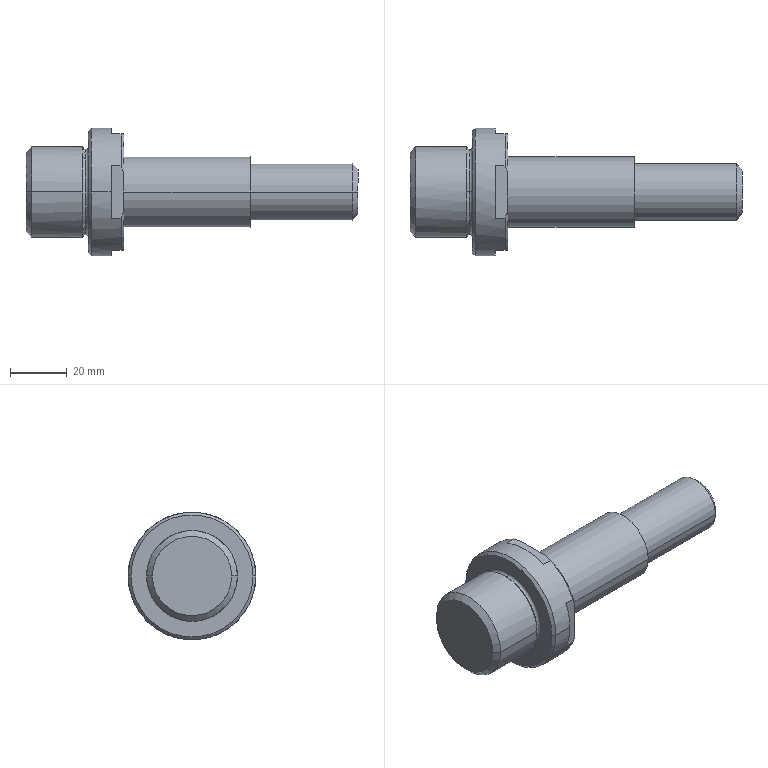Component | SolidWorks | FE5-225--a_b-1 | 1 solid | 35 faces | box 117 x 45 x 45 mm | volume 70338 mm3 | plane 13 | cone 10 | cylinder 8 | torus 4 | commonest cylinder face diameters 32 x2 20 x2 25 x2 45 x2
build123d program:
from build123d import *

# Parameters (mm, degrees)
SKETCH2_R       = 1
CHAMFER2_1_SIZE = 2
CHAMFER1_1_SIZE = 1
SKETCH3_W       = 30
SKETCH3_H       = 5
SKETCH3_W_2     = 5
SKETCH3_H_2     = 30
EXTRUDE1_DEPTH  = 4.5


with BuildPart() as part:
    # Sketch1 → Revolve1 (revolve)
    with BuildSketch(Plane(origin=(0, 0, 0), x_dir=(0, 0, -1), z_dir=(1, 0, 0))):
        Polygon((-117, 0), (-117, 16), (-95, 16), (-95, 22.5), (-82.5, 22.5), (-82.5, 12.5), (-38, 12.5), (-38, 10), (0, 10), (0, 0), align=None)
    revolve(axis=Axis((0, 0, 0), (0, 0, 1)))

    # Sketch2 → Cut-Revolve1 (revolve, cut)
    with BuildSketch(Plane(origin=(0, 0, 0), x_dir=(0, 0, -1), z_dir=(1, 0, 0)), mode=Mode.PRIVATE) as cut_revolve1_sk:
        with Locations((-96, 16)):
            Circle(SKETCH2_R)
    revolve(cut_revolve1_sk.sketch.rotate(Axis((0, 0, 0), (0, 0, 1)), 90), axis=Axis((0, 0, 0), (0, 0, 1)), mode=Mode.SUBTRACT)

    # Chamfer2-1
    chamfer2_1_edges = [part.edges().sort_by_distance(p)[0] for p in [
        (0, -16, 117),
        (0, -10, 0),
    ]]
    chamfer(chamfer2_1_edges, length=CHAMFER2_1_SIZE)

    # Chamfer1-1
    chamfer1_1_edges = [part.edges().sort_by_distance(p)[0] for p in [
        (0, -22.5, 82.5),
        (0, -22.5, 95),
    ]]
    chamfer(chamfer1_1_edges, length=CHAMFER1_1_SIZE)

    # Sketch3 → Extrude1 (cut)
    with BuildSketch(Plane(origin=(0, 0, 82.5), x_dir=(-1, 0, 0), z_dir=(0, 0, -1))):
        with Locations((0, 23)):
            Rectangle(SKETCH3_W, SKETCH3_H)
        with Locations((23, 0)):
            Rectangle(SKETCH3_W_2, SKETCH3_H_2)
        with Locations((-23, 0)):
            Rectangle(SKETCH3_W_2, SKETCH3_H_2)
        with Locations((0, -23)):
            Rectangle(SKETCH3_W, SKETCH3_H)
    extrude(amount=-EXTRUDE1_DEPTH, mode=Mode.SUBTRACT)


solid = part.part

# Placed as in the assembly
solid = solid.moved(Location((102, 81, -524), (0, -90, 0)))
STEP:
#1=COLOUR_RGB('',0.7922,0.8196,0.9333);
#2=FILL_AREA_STYLE_COLOUR('',#1);
#3=FILL_AREA_STYLE('',(#2));
#4=SURFACE_STYLE_FILL_AREA(#3);
#5=SURFACE_SIDE_STYLE('',(#4));
#6=SURFACE_STYLE_USAGE(.BOTH.,#5);
#7=PRESENTATION_STYLE_ASSIGNMENT((#6));
#8=CARTESIAN_POINT('',(0.2756,3.189,-21.26));
#9=VERTEX_POINT('',#8);
#10=CARTESIAN_POINT('',(0.2362,3.189,-21.22));
#11=VERTEX_POINT('',#10);
#12=CARTESIAN_POINT('',(0.2362,3.189,-21.26));
#13=DIRECTION('',(-0.,-1.,-0.));
#14=DIRECTION('',(1.,0.,0.));
#15=AXIS2_PLACEMENT_3D('',#12,#13,#14);
#16=CIRCLE('',#15,0.03937);
#17=EDGE_CURVE('',#9,#11,#16,.T.);
#18=ORIENTED_EDGE('',*,*,#17,.T.);
#19=CARTESIAN_POINT('',(0.2362,3.189,-20.039));
#20=VERTEX_POINT('',#19);
#21=CARTESIAN_POINT('',(0.2362,3.189,-20.63));
#22=DIRECTION('',(1.,-0.,-0.));
#23=DIRECTION('',(-0.,0.,-1.));
#24=AXIS2_PLACEMENT_3D('',#21,#22,#23);
#25=CIRCLE('',#24,0.5906);
#26=EDGE_CURVE('',#11,#20,#25,.T.);
#27=ORIENTED_EDGE('',*,*,#26,.T.);
#28=CARTESIAN_POINT('',(0.2756,3.189,-20.));
#29=VERTEX_POINT('',#28);
#30=CARTESIAN_POINT('',(0.2362,3.189,-20.));
#31=DIRECTION('',(0.,1.,-0.));
#32=DIRECTION('',(-1.,0.,0.));
#33=AXIS2_PLACEMENT_3D('',#30,#31,#32);
#34=CIRCLE('',#33,0.03937);
#35=EDGE_CURVE('',#29,#20,#34,.T.);
#36=ORIENTED_EDGE('',*,*,#35,.F.);
#37=CARTESIAN_POINT('',(0.2756,3.189,-20.63));
#38=DIRECTION('',(1.,-0.,-0.));
#39=DIRECTION('',(-0.,0.,-1.));
#40=AXIS2_PLACEMENT_3D('',#37,#38,#39);
#41=CIRCLE('',#40,0.6299);
#42=EDGE_CURVE('',#9,#29,#41,.T.);
#43=ORIENTED_EDGE('',*,*,#42,.F.);
#44=EDGE_LOOP('',(#18,#27,#36,#43));
#45=FACE_OUTER_BOUND('',#44,.T.);
#46=CARTESIAN_POINT('',(0.2362,3.189,-20.63));
#47=DIRECTION('',(1.,-0.,-0.));
#48=DIRECTION('',(-0.,0.,-1.));
#49=AXIS2_PLACEMENT_3D('',#46,#47,#48);
#50=TOROIDAL_SURFACE('',#49,0.6299,0.03937);
#51=ADVANCED_FACE('',(#45),#50,.F.);
#52=ORIENTED_EDGE('',*,*,#35,.T.);
#53=CARTESIAN_POINT('',(0.2362,3.189,-20.63));
#54=DIRECTION('',(1.,-0.,-0.));
#55=DIRECTION('',(-0.,0.,-1.));
#56=AXIS2_PLACEMENT_3D('',#53,#54,#55);
#57=CIRCLE('',#56,0.5906);
#58=EDGE_CURVE('',#20,#11,#57,.T.);
#59=ORIENTED_EDGE('',*,*,#58,.T.);
#60=ORIENTED_EDGE('',*,*,#17,.F.);
#61=CARTESIAN_POINT('',(0.2756,3.189,-20.63));
#62=DIRECTION('',(1.,-0.,-0.));
#63=DIRECTION('',(-0.,0.,-1.));
#64=AXIS2_PLACEMENT_3D('',#61,#62,#63);
#65=CIRCLE('',#64,0.6299);
#66=EDGE_CURVE('',#29,#9,#65,.T.);
#67=ORIENTED_EDGE('',*,*,#66,.F.);
#68=EDGE_LOOP('',(#52,#59,#60,#67));
#69=FACE_OUTER_BOUND('',#68,.T.);
#70=CARTESIAN_POINT('',(0.2362,3.189,-20.63));
#71=DIRECTION('',(1.,-0.,-0.));
#72=DIRECTION('',(-0.,0.,-1.));
#73=AXIS2_PLACEMENT_3D('',#70,#71,#72);
#74=TOROIDAL_SURFACE('',#73,0.6299,0.03937);
#75=ADVANCED_FACE('',(#69),#74,.F.);
#76=CARTESIAN_POINT('',(0.2756,2.343,-20.63));
#77=VERTEX_POINT('',#76);
#78=CARTESIAN_POINT('',(0.2756,4.035,-20.63));
#79=VERTEX_POINT('',#78);
#80=CARTESIAN_POINT('',(0.2756,3.189,-20.63));
#81=DIRECTION('',(-1.,0.,0.));
#82=DIRECTION('',(0.,-1.,0.));
#83=AXIS2_PLACEMENT_3D('',#80,#81,#82);
#84=CIRCLE('',#83,0.8465);
#85=EDGE_CURVE('',#77,#79,#84,.T.);
#86=ORIENTED_EDGE('',*,*,#85,.F.);
#87=CARTESIAN_POINT('',(0.315,2.303,-20.63));
#88=VERTEX_POINT('',#87);
#89=CARTESIAN_POINT('',(0.315,2.303,-20.63));
#90=DIRECTION('',(0.7071,-0.7071,-0.));
#91=VECTOR('',#90,39.37);
#92=LINE('',#89,#91);
#93=EDGE_CURVE('',#77,#88,#92,.T.);
#94=ORIENTED_EDGE('',*,*,#93,.T.);
#95=CARTESIAN_POINT('',(0.315,4.075,-20.63));
#96=VERTEX_POINT('',#95);
#97=CARTESIAN_POINT('',(0.315,3.189,-20.63));
#98=DIRECTION('',(1.,0.,-0.));
#99=DIRECTION('',(0.,-1.,0.));
#100=AXIS2_PLACEMENT_3D('',#97,#98,#99);
#101=CIRCLE('',#100,0.8858);
#102=EDGE_CURVE('',#96,#88,#101,.T.);
#103=ORIENTED_EDGE('',*,*,#102,.F.);
#104=CARTESIAN_POINT('',(0.315,4.075,-20.63));
#105=DIRECTION('',(0.7071,0.7071,-0.));
#106=VECTOR('',#105,39.37);
#107=LINE('',#104,#106);
#108=EDGE_CURVE('',#79,#96,#107,.T.);
#109=ORIENTED_EDGE('',*,*,#108,.F.);
#110=EDGE_LOOP('',(#86,#94,#103,#109));
#111=FACE_OUTER_BOUND('',#110,.T.);
#112=CARTESIAN_POINT('',(0.315,3.189,-20.63));
#113=DIRECTION('',(1.,0.,-0.));
#114=DIRECTION('',(0.,1.,0.));
#115=AXIS2_PLACEMENT_3D('',#112,#113,#114);
#116=CONICAL_SURFACE('',#115,0.8858,0.7854);
#117=ADVANCED_FACE('',(#111),#116,.T.);
#118=CARTESIAN_POINT('',(-0.5906,2.638,-20.63));
#119=VERTEX_POINT('',#118);
#120=CARTESIAN_POINT('',(-0.5906,3.74,-20.63));
#121=VERTEX_POINT('',#120);
#122=CARTESIAN_POINT('',(-0.5906,3.189,-20.63));
#123=DIRECTION('',(-1.,0.,0.));
#124=DIRECTION('',(0.,-1.,0.));
#125=AXIS2_PLACEMENT_3D('',#122,#123,#124);
#126=CIRCLE('',#125,0.5512);
#127=EDGE_CURVE('',#119,#121,#126,.T.);
#128=ORIENTED_EDGE('',*,*,#127,.F.);
#129=CARTESIAN_POINT('',(-0.5118,2.559,-20.63));
#130=VERTEX_POINT('',#129);
#131=CARTESIAN_POINT('',(-0.5118,2.559,-20.63));
#132=DIRECTION('',(0.7071,-0.7071,-0.));
#133=VECTOR('',#132,39.37);
#134=LINE('',#131,#133);
#135=EDGE_CURVE('',#119,#130,#134,.T.);
#136=ORIENTED_EDGE('',*,*,#135,.T.);
#137=CARTESIAN_POINT('',(-0.5118,3.819,-20.63));
#138=VERTEX_POINT('',#137);
#139=CARTESIAN_POINT('',(-0.5118,3.189,-20.63));
#140=DIRECTION('',(1.,0.,-0.));
#141=DIRECTION('',(0.,-1.,0.));
#142=AXIS2_PLACEMENT_3D('',#139,#140,#141);
#143=CIRCLE('',#142,0.6299);
#144=EDGE_CURVE('',#138,#130,#143,.T.);
#145=ORIENTED_EDGE('',*,*,#144,.F.);
#146=CARTESIAN_POINT('',(-0.5118,3.819,-20.63));
#147=DIRECTION('',(0.7071,0.7071,-0.));
#148=VECTOR('',#147,39.37);
#149=LINE('',#146,#148);
#150=EDGE_CURVE('',#121,#138,#149,.T.);
#151=ORIENTED_EDGE('',*,*,#150,.F.);
#152=EDGE_LOOP('',(#128,#136,#145,#151));
#153=FACE_OUTER_BOUND('',#152,.T.);
#154=CARTESIAN_POINT('',(-0.5118,3.189,-20.63));
#155=DIRECTION('',(1.,0.,-0.));
#156=DIRECTION('',(0.,1.,0.));
#157=AXIS2_PLACEMENT_3D('',#154,#155,#156);
#158=CONICAL_SURFACE('',#157,0.6299,0.7854);
#159=ADVANCED_FACE('',(#153),#158,.T.);
#160=CARTESIAN_POINT('',(4.016,3.504,-20.63));
#161=VERTEX_POINT('',#160);
#162=CARTESIAN_POINT('',(4.016,2.874,-20.63));
#163=VERTEX_POINT('',#162);
#164=CARTESIAN_POINT('',(4.016,3.189,-20.63));
#165=DIRECTION('',(1.,-0.,-0.));
#166=DIRECTION('',(0.,1.,0.));
#167=AXIS2_PLACEMENT_3D('',#164,#165,#166);
#168=CIRCLE('',#167,0.315);
#169=EDGE_CURVE('',#161,#163,#168,.T.);
#170=ORIENTED_EDGE('',*,*,#169,.F.);
#171=CARTESIAN_POINT('',(3.937,3.583,-20.63));
#172=VERTEX_POINT('',#171);
#173=CARTESIAN_POINT('',(4.016,3.504,-20.63));
#174=DIRECTION('',(-0.7071,0.7071,0.));
#175=VECTOR('',#174,39.37);
#176=LINE('',#173,#175);
#177=EDGE_CURVE('',#161,#172,#176,.T.);
#178=ORIENTED_EDGE('',*,*,#177,.T.);
#179=CARTESIAN_POINT('',(3.937,2.795,-20.63));
#180=VERTEX_POINT('',#179);
#181=CARTESIAN_POINT('',(3.937,3.189,-20.63));
#182=DIRECTION('',(-1.,0.,0.));
#183=DIRECTION('',(0.,1.,0.));
#184=AXIS2_PLACEMENT_3D('',#181,#182,#183);
#185=CIRCLE('',#184,0.3937);
#186=EDGE_CURVE('',#180,#172,#185,.T.);
#187=ORIENTED_EDGE('',*,*,#186,.F.);
#188=CARTESIAN_POINT('',(4.016,2.874,-20.63));
#189=DIRECTION('',(-0.7071,-0.7071,0.));
#190=VECTOR('',#189,39.37);
#191=LINE('',#188,#190);
#192=EDGE_CURVE('',#163,#180,#191,.T.);
#193=ORIENTED_EDGE('',*,*,#192,.F.);
#194=EDGE_LOOP('',(#170,#178,#187,#193));
#195=FACE_OUTER_BOUND('',#194,.T.);
#196=CARTESIAN_POINT('',(4.016,3.189,-20.63));
#197=DIRECTION('',(-1.,0.,0.));
#198=DIRECTION('',(0.,-1.,0.));
#199=AXIS2_PLACEMENT_3D('',#196,#197,#198);
#200=CONICAL_SURFACE('',#199,0.315,0.7854);
#201=ADVANCED_FACE('',(#195),#200,.T.);
#202=ORIENTED_EDGE('',*,*,#144,.T.);
#203=CARTESIAN_POINT('',(0.1969,2.559,-20.63));
#204=VERTEX_POINT('',#203);
#205=CARTESIAN_POINT('',(4.016,2.559,-20.63));
#206=DIRECTION('',(1.,-0.,-0.));
#207=VECTOR('',#206,39.37);
#208=LINE('',#205,#207);
#209=EDGE_CURVE('',#130,#204,#208,.T.);
#210=ORIENTED_EDGE('',*,*,#209,.T.);
#211=CARTESIAN_POINT('',(0.1969,3.189,-20.));
#212=VERTEX_POINT('',#211);
#213=CARTESIAN_POINT('',(0.1969,3.189,-20.63));
#214=DIRECTION('',(1.,-0.,-0.));
#215=DIRECTION('',(-0.,0.,-1.));
#216=AXIS2_PLACEMENT_3D('',#213,#214,#215);
#217=CIRCLE('',#216,0.6299);
#218=EDGE_CURVE('',#212,#204,#217,.T.);
#219=ORIENTED_EDGE('',*,*,#218,.F.);
#220=CARTESIAN_POINT('',(0.1969,3.819,-20.63));
#221=VERTEX_POINT('',#220);
#222=CARTESIAN_POINT('',(0.1969,3.189,-20.63));
#223=DIRECTION('',(1.,-0.,-0.));
#224=DIRECTION('',(-0.,0.,-1.));
#225=AXIS2_PLACEMENT_3D('',#222,#223,#224);
#226=CIRCLE('',#225,0.6299);
#227=EDGE_CURVE('',#221,#212,#226,.T.);
#228=ORIENTED_EDGE('',*,*,#227,.F.);
#229=CARTESIAN_POINT('',(4.016,3.819,-20.63));
#230=DIRECTION('',(1.,-0.,-0.));
#231=VECTOR('',#230,39.37);
#232=LINE('',#229,#231);
#233=EDGE_CURVE('',#138,#221,#232,.T.);
#234=ORIENTED_EDGE('',*,*,#233,.F.);
#235=EDGE_LOOP('',(#202,#210,#219,#228,#234));
#236=FACE_OUTER_BOUND('',#235,.T.);
#237=CARTESIAN_POINT('',(4.016,3.189,-20.63));
#238=DIRECTION('',(1.,-0.,-0.));
#239=DIRECTION('',(0.,1.,0.));
#240=AXIS2_PLACEMENT_3D('',#237,#238,#239);
#241=CYLINDRICAL_SURFACE('',#240,0.6299);
#242=ADVANCED_FACE('',(#236),#241,.T.);
#243=ORIENTED_EDGE('',*,*,#58,.F.);
#244=CARTESIAN_POINT('',(0.2362,3.189,-20.));
#245=DIRECTION('',(0.,1.,-0.));
#246=DIRECTION('',(-1.,0.,0.));
#247=AXIS2_PLACEMENT_3D('',#244,#245,#246);
#248=CIRCLE('',#247,0.03937);
#249=EDGE_CURVE('',#20,#212,#248,.T.);
#250=ORIENTED_EDGE('',*,*,#249,.T.);
#251=ORIENTED_EDGE('',*,*,#218,.T.);
#252=CARTESIAN_POINT('',(0.1969,3.189,-21.26));
#253=VERTEX_POINT('',#252);
#254=CARTESIAN_POINT('',(0.1969,3.189,-20.63));
#255=DIRECTION('',(1.,-0.,-0.));
#256=DIRECTION('',(-0.,0.,-1.));
#257=AXIS2_PLACEMENT_3D('',#254,#255,#256);
#258=CIRCLE('',#257,0.6299);
#259=EDGE_CURVE('',#204,#253,#258,.T.);
#260=ORIENTED_EDGE('',*,*,#259,.T.);
#261=CARTESIAN_POINT('',(0.2362,3.189,-21.26));
#262=DIRECTION('',(-0.,-1.,-0.));
#263=DIRECTION('',(1.,0.,0.));
#264=AXIS2_PLACEMENT_3D('',#261,#262,#263);
#265=CIRCLE('',#264,0.03937);
#266=EDGE_CURVE('',#11,#253,#265,.T.);
#267=ORIENTED_EDGE('',*,*,#266,.F.);
#268=EDGE_LOOP('',(#243,#250,#251,#260,#267));
#269=FACE_OUTER_BOUND('',#268,.T.);
#270=CARTESIAN_POINT('',(0.2362,3.189,-20.63));
#271=DIRECTION('',(1.,-0.,-0.));
#272=DIRECTION('',(-0.,0.,-1.));
#273=AXIS2_PLACEMENT_3D('',#270,#271,#272);
#274=TOROIDAL_SURFACE('',#273,0.6299,0.03937);
#275=ADVANCED_FACE('',(#269),#274,.F.);
#276=CARTESIAN_POINT('',(2.52,3.583,-20.63));
#277=VERTEX_POINT('',#276);
#278=CARTESIAN_POINT('',(2.52,2.795,-20.63));
#279=VERTEX_POINT('',#278);
#280=CARTESIAN_POINT('',(2.52,3.189,-20.63));
#281=DIRECTION('',(1.,-0.,-0.));
#282=DIRECTION('',(0.,1.,0.));
#283=AXIS2_PLACEMENT_3D('',#280,#281,#282);
#284=CIRCLE('',#283,0.3937);
#285=EDGE_CURVE('',#277,#279,#284,.T.);
#286=ORIENTED_EDGE('',*,*,#285,.T.);
#287=CARTESIAN_POINT('',(4.016,2.795,-20.63));
#288=DIRECTION('',(1.,-0.,-0.));
#289=VECTOR('',#288,39.37);
#290=LINE('',#287,#289);
#291=EDGE_CURVE('',#279,#180,#290,.T.);
#292=ORIENTED_EDGE('',*,*,#291,.T.);
#293=ORIENTED_EDGE('',*,*,#186,.T.);
#294=CARTESIAN_POINT('',(4.016,3.583,-20.63));
#295=DIRECTION('',(1.,-0.,-0.));
#296=VECTOR('',#295,39.37);
#297=LINE('',#294,#296);
#298=EDGE_CURVE('',#277,#172,#297,.T.);
#299=ORIENTED_EDGE('',*,*,#298,.F.);
#300=EDGE_LOOP('',(#286,#292,#293,#299));
#301=FACE_OUTER_BOUND('',#300,.T.);
#302=CARTESIAN_POINT('',(4.016,3.189,-20.63));
#303=DIRECTION('',(1.,-0.,-0.));
#304=DIRECTION('',(0.,1.,0.));
#305=AXIS2_PLACEMENT_3D('',#302,#303,#304);
#306=CYLINDRICAL_SURFACE('',#305,0.3937);
#307=ADVANCED_FACE('',(#301),#306,.T.);
#308=CARTESIAN_POINT('',(0.7677,3.681,-20.63));
#309=VERTEX_POINT('',#308);
#310=CARTESIAN_POINT('',(0.7677,2.697,-20.63));
#311=VERTEX_POINT('',#310);
#312=CARTESIAN_POINT('',(0.7677,3.189,-20.63));
#313=DIRECTION('',(1.,-0.,-0.));
#314=DIRECTION('',(0.,1.,0.));
#315=AXIS2_PLACEMENT_3D('',#312,#313,#314);
#316=CIRCLE('',#315,0.4921);
#317=EDGE_CURVE('',#309,#311,#316,.T.);
#318=ORIENTED_EDGE('',*,*,#317,.T.);
#319=CARTESIAN_POINT('',(2.52,2.697,-20.63));
#320=VERTEX_POINT('',#319);
#321=CARTESIAN_POINT('',(4.016,2.697,-20.63));
#322=DIRECTION('',(1.,-0.,-0.));
#323=VECTOR('',#322,39.37);
#324=LINE('',#321,#323);
#325=EDGE_CURVE('',#311,#320,#324,.T.);
#326=ORIENTED_EDGE('',*,*,#325,.T.);
#327=CARTESIAN_POINT('',(2.52,3.681,-20.63));
#328=VERTEX_POINT('',#327);
#329=CARTESIAN_POINT('',(2.52,3.189,-20.63));
#330=DIRECTION('',(1.,-0.,-0.));
#331=DIRECTION('',(0.,1.,0.));
#332=AXIS2_PLACEMENT_3D('',#329,#330,#331);
#333=CIRCLE('',#332,0.4921);
#334=EDGE_CURVE('',#328,#320,#333,.T.);
#335=ORIENTED_EDGE('',*,*,#334,.F.);
#336=CARTESIAN_POINT('',(4.016,3.681,-20.63));
#337=DIRECTION('',(1.,-0.,-0.));
#338=VECTOR('',#337,39.37);
#339=LINE('',#336,#338);
#340=EDGE_CURVE('',#309,#328,#339,.T.);
#341=ORIENTED_EDGE('',*,*,#340,.F.);
#342=EDGE_LOOP('',(#318,#326,#335,#341));
#343=FACE_OUTER_BOUND('',#342,.T.);
#344=CARTESIAN_POINT('',(4.016,3.189,-20.63));
#345=DIRECTION('',(1.,-0.,-0.));
#346=DIRECTION('',(0.,1.,0.));
#347=AXIS2_PLACEMENT_3D('',#344,#345,#346);
#348=CYLINDRICAL_SURFACE('',#347,0.4921);
#349=ADVANCED_FACE('',(#343),#348,.T.);
#350=ORIENTED_EDGE('',*,*,#102,.T.);
#351=CARTESIAN_POINT('',(0.5906,2.303,-20.63));
#352=VERTEX_POINT('',#351);
#353=CARTESIAN_POINT('',(4.016,2.303,-20.63));
#354=DIRECTION('',(1.,-0.,-0.));
#355=VECTOR('',#354,39.37);
#356=LINE('',#353,#355);
#357=EDGE_CURVE('',#88,#352,#356,.T.);
#358=ORIENTED_EDGE('',*,*,#357,.T.);
#359=CARTESIAN_POINT('',(0.5906,2.382,-20.265));
#360=VERTEX_POINT('',#359);
#361=CARTESIAN_POINT('',(0.5906,3.189,-20.63));
#362=DIRECTION('',(-1.,0.,0.));
#363=DIRECTION('',(-0.,0.,-1.));
#364=AXIS2_PLACEMENT_3D('',#361,#362,#363);
#365=CIRCLE('',#364,0.8858);
#366=EDGE_CURVE('',#352,#360,#365,.T.);
#367=ORIENTED_EDGE('',*,*,#366,.T.);
#368=CARTESIAN_POINT('',(0.7283,2.382,-20.265));
#369=VERTEX_POINT('',#368);
#370=CARTESIAN_POINT('',(4.016,2.382,-20.265));
#371=DIRECTION('',(-1.,0.,0.));
#372=VECTOR('',#371,39.37);
#373=LINE('',#370,#372);
#374=EDGE_CURVE('',#369,#360,#373,.T.);
#375=ORIENTED_EDGE('',*,*,#374,.F.);
#376=CARTESIAN_POINT('',(0.7283,2.824,-19.823));
#377=VERTEX_POINT('',#376);
#378=CARTESIAN_POINT('',(0.7283,3.189,-20.63));
#379=DIRECTION('',(-1.,0.,0.));
#380=DIRECTION('',(0.,1.,0.));
#381=AXIS2_PLACEMENT_3D('',#378,#379,#380);
#382=CIRCLE('',#381,0.8858);
#383=EDGE_CURVE('',#369,#377,#382,.T.);
#384=ORIENTED_EDGE('',*,*,#383,.T.);
#385=CARTESIAN_POINT('',(0.5906,2.824,-19.823));
#386=VERTEX_POINT('',#385);
#387=CARTESIAN_POINT('',(4.016,2.824,-19.823));
#388=DIRECTION('',(1.,-0.,-0.));
#389=VECTOR('',#388,39.37);
#390=LINE('',#387,#389);
#391=EDGE_CURVE('',#386,#377,#390,.T.);
#392=ORIENTED_EDGE('',*,*,#391,.F.);
#393=CARTESIAN_POINT('',(0.5906,3.554,-19.823));
#394=VERTEX_POINT('',#393);
#395=CARTESIAN_POINT('',(0.5906,3.189,-20.63));
#396=DIRECTION('',(-1.,0.,0.));
#397=DIRECTION('',(-0.,-0.,-1.));
#398=AXIS2_PLACEMENT_3D('',#395,#396,#397);
#399=CIRCLE('',#398,0.8858);
#400=EDGE_CURVE('',#386,#394,#399,.T.);
#401=ORIENTED_EDGE('',*,*,#400,.T.);
#402=CARTESIAN_POINT('',(0.7283,3.554,-19.823));
#403=VERTEX_POINT('',#402);
#404=CARTESIAN_POINT('',(4.016,3.554,-19.823));
#405=DIRECTION('',(-1.,0.,0.));
#406=VECTOR('',#405,39.37);
#407=LINE('',#404,#406);
#408=EDGE_CURVE('',#403,#394,#407,.T.);
#409=ORIENTED_EDGE('',*,*,#408,.F.);
#410=CARTESIAN_POINT('',(0.7283,3.996,-20.265));
#411=VERTEX_POINT('',#410);
#412=CARTESIAN_POINT('',(0.7283,3.189,-20.63));
#413=DIRECTION('',(-1.,0.,0.));
#414=DIRECTION('',(0.,1.,0.));
#415=AXIS2_PLACEMENT_3D('',#412,#413,#414);
#416=CIRCLE('',#415,0.8858);
#417=EDGE_CURVE('',#403,#411,#416,.T.);
#418=ORIENTED_EDGE('',*,*,#417,.T.);
#419=CARTESIAN_POINT('',(0.5906,3.996,-20.265));
#420=VERTEX_POINT('',#419);
#421=CARTESIAN_POINT('',(4.016,3.996,-20.265));
#422=DIRECTION('',(1.,-0.,-0.));
#423=VECTOR('',#422,39.37);
#424=LINE('',#421,#423);
#425=EDGE_CURVE('',#420,#411,#424,.T.);
#426=ORIENTED_EDGE('',*,*,#425,.F.);
#427=CARTESIAN_POINT('',(0.5906,4.075,-20.63));
#428=VERTEX_POINT('',#427);
#429=CARTESIAN_POINT('',(0.5906,3.189,-20.63));
#430=DIRECTION('',(-1.,0.,0.));
#431=DIRECTION('',(-0.,0.,-1.));
#432=AXIS2_PLACEMENT_3D('',#429,#430,#431);
#433=CIRCLE('',#432,0.8858);
#434=EDGE_CURVE('',#420,#428,#433,.T.);
#435=ORIENTED_EDGE('',*,*,#434,.T.);
#436=CARTESIAN_POINT('',(4.016,4.075,-20.63));
#437=DIRECTION('',(1.,-0.,-0.));
#438=VECTOR('',#437,39.37);
#439=LINE('',#436,#438);
#440=EDGE_CURVE('',#96,#428,#439,.T.);
#441=ORIENTED_EDGE('',*,*,#440,.F.);
#442=EDGE_LOOP('',(#350,#358,#367,#375,#384,#392,#401,#409,#418,#426,#435,#441));
#443=FACE_OUTER_BOUND('',#442,.T.);
#444=CARTESIAN_POINT('',(4.016,3.189,-20.63));
#445=DIRECTION('',(1.,-0.,-0.));
#446=DIRECTION('',(0.,1.,0.));
#447=AXIS2_PLACEMENT_3D('',#444,#445,#446);
#448=CYLINDRICAL_SURFACE('',#447,0.8858);
#449=ADVANCED_FACE('',(#443),#448,.T.);
#450=CARTESIAN_POINT('',(0.7283,2.382,-20.995));
#451=VERTEX_POINT('',#450);
#452=CARTESIAN_POINT('',(0.7677,2.382,-20.885));
#453=VERTEX_POINT('',#452);
#454=CARTESIAN_POINT('',(0.7283,2.382,-20.995));
#455=CARTESIAN_POINT('',(0.7431,2.382,-20.959));
#456=CARTESIAN_POINT('',(0.7564,2.382,-20.923));
#457=CARTESIAN_POINT('',(0.7677,2.382,-20.885));
#458=B_SPLINE_CURVE_WITH_KNOTS('',3,(#454,#455,#456,#457),.UNSPECIFIED.,.F.,.F.,(4,4),(0.02898,0.03193),.UNSPECIFIED.);
#459=EDGE_CURVE('',#451,#453,#458,.T.);
#460=ORIENTED_EDGE('',*,*,#459,.F.);
#461=CARTESIAN_POINT('',(0.7283,2.824,-21.437));
#462=VERTEX_POINT('',#461);
#463=CARTESIAN_POINT('',(0.7283,3.189,-20.63));
#464=DIRECTION('',(-1.,0.,0.));
#465=DIRECTION('',(0.,1.,0.));
#466=AXIS2_PLACEMENT_3D('',#463,#464,#465);
#467=CIRCLE('',#466,0.8858);
#468=EDGE_CURVE('',#462,#451,#467,.T.);
#469=ORIENTED_EDGE('',*,*,#468,.F.);
#470=CARTESIAN_POINT('',(0.7677,2.934,-21.437));
#471=VERTEX_POINT('',#470);
#472=CARTESIAN_POINT('',(0.7677,2.934,-21.437));
#473=CARTESIAN_POINT('',(0.7565,2.897,-21.437));
#474=CARTESIAN_POINT('',(0.7433,2.86,-21.437));
#475=CARTESIAN_POINT('',(0.7283,2.824,-21.437));
#476=B_SPLINE_CURVE_WITH_KNOTS('',3,(#472,#473,#474,#475),.UNSPECIFIED.,.F.,.F.,(4,4),(0.04504,0.04799),.UNSPECIFIED.);
#477=EDGE_CURVE('',#471,#462,#476,.T.);
#478=ORIENTED_EDGE('',*,*,#477,.F.);
#479=CARTESIAN_POINT('',(0.7677,3.189,-20.63));
#480=DIRECTION('',(1.,-0.,-0.));
#481=DIRECTION('',(0.,1.,0.));
#482=AXIS2_PLACEMENT_3D('',#479,#480,#481);
#483=CIRCLE('',#482,0.8465);
#484=EDGE_CURVE('',#453,#471,#483,.T.);
#485=ORIENTED_EDGE('',*,*,#484,.F.);
#486=EDGE_LOOP('',(#460,#469,#478,#485));
#487=FACE_OUTER_BOUND('',#486,.T.);
#488=CARTESIAN_POINT('',(0.7677,3.189,-20.63));
#489=DIRECTION('',(-1.,0.,0.));
#490=DIRECTION('',(0.,-1.,0.));
#491=AXIS2_PLACEMENT_3D('',#488,#489,#490);
#492=CONICAL_SURFACE('',#491,0.8465,0.7854);
#493=ADVANCED_FACE('',(#487),#492,.T.);
#494=CARTESIAN_POINT('',(0.7677,2.382,-20.375));
#495=VERTEX_POINT('',#494);
#496=CARTESIAN_POINT('',(0.7677,2.382,-20.375));
#497=CARTESIAN_POINT('',(0.7565,2.382,-20.338));
#498=CARTESIAN_POINT('',(0.7433,2.382,-20.301));
#499=CARTESIAN_POINT('',(0.7283,2.382,-20.265));
#500=B_SPLINE_CURVE_WITH_KNOTS('',3,(#496,#497,#498,#499),.UNSPECIFIED.,.F.,.F.,(4,4),(0.04504,0.04799),.UNSPECIFIED.);
#501=EDGE_CURVE('',#495,#369,#500,.T.);
#502=ORIENTED_EDGE('',*,*,#501,.F.);
#503=CARTESIAN_POINT('',(0.7677,2.934,-19.823));
#504=VERTEX_POINT('',#503);
#505=CARTESIAN_POINT('',(0.7677,3.189,-20.63));
#506=DIRECTION('',(1.,-0.,-0.));
#507=DIRECTION('',(0.,1.,0.));
#508=AXIS2_PLACEMENT_3D('',#505,#506,#507);
#509=CIRCLE('',#508,0.8465);
#510=EDGE_CURVE('',#504,#495,#509,.T.);
#511=ORIENTED_EDGE('',*,*,#510,.F.);
#512=CARTESIAN_POINT('',(0.7283,2.824,-19.823));
#513=CARTESIAN_POINT('',(0.7431,2.86,-19.823));
#514=CARTESIAN_POINT('',(0.7564,2.896,-19.823));
#515=CARTESIAN_POINT('',(0.7677,2.934,-19.823));
#516=B_SPLINE_CURVE_WITH_KNOTS('',3,(#512,#513,#514,#515),.UNSPECIFIED.,.F.,.F.,(4,4),(0.02898,0.03193),.UNSPECIFIED.);
#517=EDGE_CURVE('',#377,#504,#516,.T.);
#518=ORIENTED_EDGE('',*,*,#517,.F.);
#519=ORIENTED_EDGE('',*,*,#383,.F.);
#520=EDGE_LOOP('',(#502,#511,#518,#519));
#521=FACE_OUTER_BOUND('',#520,.T.);
#522=CARTESIAN_POINT('',(0.7677,3.189,-20.63));
#523=DIRECTION('',(-1.,0.,0.));
#524=DIRECTION('',(0.,-1.,0.));
#525=AXIS2_PLACEMENT_3D('',#522,#523,#524);
#526=CONICAL_SURFACE('',#525,0.8465,0.7854);
#527=ADVANCED_FACE('',(#521),#526,.T.);
#528=CARTESIAN_POINT('',(0.7283,3.554,-21.437));
#529=VERTEX_POINT('',#528);
#530=CARTESIAN_POINT('',(0.7677,3.444,-21.437));
#531=VERTEX_POINT('',#530);
#532=CARTESIAN_POINT('',(0.7283,3.554,-21.437));
#533=CARTESIAN_POINT('',(0.7431,3.518,-21.437));
#534=CARTESIAN_POINT('',(0.7564,3.482,-21.437));
#535=CARTESIAN_POINT('',(0.7677,3.444,-21.437));
#536=B_SPLINE_CURVE_WITH_KNOTS('',3,(#532,#533,#534,#535),.UNSPECIFIED.,.F.,.F.,(4,4),(0.02898,0.03193),.UNSPECIFIED.);
#537=EDGE_CURVE('',#529,#531,#536,.T.);
#538=ORIENTED_EDGE('',*,*,#537,.F.);
#539=CARTESIAN_POINT('',(0.7283,3.996,-20.995));
#540=VERTEX_POINT('',#539);
#541=CARTESIAN_POINT('',(0.7283,3.189,-20.63));
#542=DIRECTION('',(-1.,0.,0.));
#543=DIRECTION('',(0.,1.,0.));
#544=AXIS2_PLACEMENT_3D('',#541,#542,#543);
#545=CIRCLE('',#544,0.8858);
#546=EDGE_CURVE('',#540,#529,#545,.T.);
#547=ORIENTED_EDGE('',*,*,#546,.F.);
#548=CARTESIAN_POINT('',(0.7677,3.996,-20.885));
#549=VERTEX_POINT('',#548);
#550=CARTESIAN_POINT('',(0.7677,3.996,-20.885));
#551=CARTESIAN_POINT('',(0.7565,3.996,-20.922));
#552=CARTESIAN_POINT('',(0.7433,3.996,-20.959));
#553=CARTESIAN_POINT('',(0.7283,3.996,-20.995));
#554=B_SPLINE_CURVE_WITH_KNOTS('',3,(#550,#551,#552,#553),.UNSPECIFIED.,.F.,.F.,(4,4),(0.04504,0.04799),.UNSPECIFIED.);
#555=EDGE_CURVE('',#549,#540,#554,.T.);
#556=ORIENTED_EDGE('',*,*,#555,.F.);
#557=CARTESIAN_POINT('',(0.7677,3.189,-20.63));
#558=DIRECTION('',(1.,-0.,-0.));
#559=DIRECTION('',(0.,1.,0.));
#560=AXIS2_PLACEMENT_3D('',#557,#558,#559);
#561=CIRCLE('',#560,0.8465);
#562=EDGE_CURVE('',#531,#549,#561,.T.);
#563=ORIENTED_EDGE('',*,*,#562,.F.);
#564=EDGE_LOOP('',(#538,#547,#556,#563));
#565=FACE_OUTER_BOUND('',#564,.T.);
#566=CARTESIAN_POINT('',(0.7677,3.189,-20.63));
#567=DIRECTION('',(-1.,0.,0.));
#568=DIRECTION('',(0.,-1.,0.));
#569=AXIS2_PLACEMENT_3D('',#566,#567,#568);
#570=CONICAL_SURFACE('',#569,0.8465,0.7854);
#571=ADVANCED_FACE('',(#565),#570,.T.);
#572=CARTESIAN_POINT('',(0.2756,3.189,-20.63));
#573=DIRECTION('',(-1.,0.,0.));
#574=DIRECTION('',(0.,-1.,0.));
#575=AXIS2_PLACEMENT_3D('',#572,#573,#574);
#576=CIRCLE('',#575,0.8465);
#577=EDGE_CURVE('',#79,#77,#576,.T.);
#578=ORIENTED_EDGE('',*,*,#577,.T.);
#579=ORIENTED_EDGE('',*,*,#85,.T.);
#580=EDGE_LOOP('',(#578,#579));
#581=FACE_OUTER_BOUND('',#580,.T.);
#582=ORIENTED_EDGE('',*,*,#42,.T.);
#583=ORIENTED_EDGE('',*,*,#66,.T.);
#584=EDGE_LOOP('',(#582,#583));
#585=FACE_BOUND('',#584,.T.);
#586=CARTESIAN_POINT('',(0.2756,3.819,-20.63));
#587=DIRECTION('',(-1.,-0.,0.));
#588=DIRECTION('',(-0.,-1.,-0.));
#589=AXIS2_PLACEMENT_3D('',#586,#587,#588);
#590=PLANE('',#589);
#591=ADVANCED_FACE('',(#581,#585),#590,.T.);
#592=ORIENTED_EDGE('',*,*,#357,.F.);
#593=CARTESIAN_POINT('',(0.315,3.189,-20.63));
#594=DIRECTION('',(1.,0.,-0.));
#595=DIRECTION('',(0.,-1.,0.));
#596=AXIS2_PLACEMENT_3D('',#593,#594,#595);
#597=CIRCLE('',#596,0.8858);
#598=EDGE_CURVE('',#88,#96,#597,.T.);
#599=ORIENTED_EDGE('',*,*,#598,.T.);
#600=ORIENTED_EDGE('',*,*,#440,.T.);
#601=CARTESIAN_POINT('',(0.5906,3.996,-20.995));
#602=VERTEX_POINT('',#601);
#603=CARTESIAN_POINT('',(0.5906,3.189,-20.63));
#604=DIRECTION('',(-1.,0.,0.));
#605=DIRECTION('',(-0.,-0.,-1.));
#606=AXIS2_PLACEMENT_3D('',#603,#604,#605);
#607=CIRCLE('',#606,0.8858);
#608=EDGE_CURVE('',#428,#602,#607,.T.);
#609=ORIENTED_EDGE('',*,*,#608,.T.);
#610=CARTESIAN_POINT('',(4.016,3.996,-20.995));
#611=DIRECTION('',(-1.,0.,0.));
#612=VECTOR('',#611,39.37);
#613=LINE('',#610,#612);
#614=EDGE_CURVE('',#540,#602,#613,.T.);
#615=ORIENTED_EDGE('',*,*,#614,.F.);
#616=ORIENTED_EDGE('',*,*,#546,.T.);
#617=CARTESIAN_POINT('',(0.5906,3.554,-21.437));
#618=VERTEX_POINT('',#617);
#619=CARTESIAN_POINT('',(4.016,3.554,-21.437));
#620=DIRECTION('',(1.,-0.,-0.));
#621=VECTOR('',#620,39.37);
#622=LINE('',#619,#621);
#623=EDGE_CURVE('',#618,#529,#622,.T.);
#624=ORIENTED_EDGE('',*,*,#623,.F.);
#625=CARTESIAN_POINT('',(0.5906,2.824,-21.437));
#626=VERTEX_POINT('',#625);
#627=CARTESIAN_POINT('',(0.5906,3.189,-20.63));
#628=DIRECTION('',(-1.,0.,0.));
#629=DIRECTION('',(-0.,-0.,-1.));
#630=AXIS2_PLACEMENT_3D('',#627,#628,#629);
#631=CIRCLE('',#630,0.8858);
#632=EDGE_CURVE('',#618,#626,#631,.T.);
#633=ORIENTED_EDGE('',*,*,#632,.T.);
#634=CARTESIAN_POINT('',(4.016,2.824,-21.437));
#635=DIRECTION('',(-1.,0.,0.));
#636=VECTOR('',#635,39.37);
#637=LINE('',#634,#636);
#638=EDGE_CURVE('',#462,#626,#637,.T.);
#639=ORIENTED_EDGE('',*,*,#638,.F.);
#640=ORIENTED_EDGE('',*,*,#468,.T.);
#641=CARTESIAN_POINT('',(0.5906,2.382,-20.995));
#642=VERTEX_POINT('',#641);
#643=CARTESIAN_POINT('',(4.016,2.382,-20.995));
#644=DIRECTION('',(1.,-0.,-0.));
#645=VECTOR('',#644,39.37);
#646=LINE('',#643,#645);
#647=EDGE_CURVE('',#642,#451,#646,.T.);
#648=ORIENTED_EDGE('',*,*,#647,.F.);
#649=CARTESIAN_POINT('',(0.5906,3.189,-20.63));
#650=DIRECTION('',(-1.,0.,0.));
#651=DIRECTION('',(-0.,-0.,-1.));
#652=AXIS2_PLACEMENT_3D('',#649,#650,#651);
#653=CIRCLE('',#652,0.8858);
#654=EDGE_CURVE('',#642,#352,#653,.T.);
#655=ORIENTED_EDGE('',*,*,#654,.T.);
#656=EDGE_LOOP('',(#592,#599,#600,#609,#615,#616,#624,#633,#639,#640,#648,#655));
#657=FACE_OUTER_BOUND('',#656,.T.);
#658=CARTESIAN_POINT('',(4.016,3.189,-20.63));
#659=DIRECTION('',(1.,-0.,-0.));
#660=DIRECTION('',(0.,1.,0.));
#661=AXIS2_PLACEMENT_3D('',#658,#659,#660);
#662=CYLINDRICAL_SURFACE('',#661,0.8858);
#663=ADVANCED_FACE('',(#657),#662,.T.);
#664=CARTESIAN_POINT('',(0.7677,2.382,-20.63));
#665=DIRECTION('',(0.,0.,1.));
#666=VECTOR('',#665,39.37);
#667=LINE('',#664,#666);
#668=EDGE_CURVE('',#453,#495,#667,.T.);
#669=ORIENTED_EDGE('',*,*,#668,.F.);
#670=ORIENTED_EDGE('',*,*,#484,.T.);
#671=CARTESIAN_POINT('',(0.7677,3.78,-21.437));
#672=DIRECTION('',(-0.,-1.,-0.));
#673=VECTOR('',#672,39.37);
#674=LINE('',#671,#673);
#675=EDGE_CURVE('',#531,#471,#674,.T.);
#676=ORIENTED_EDGE('',*,*,#675,.F.);
#677=ORIENTED_EDGE('',*,*,#562,.T.);
#678=CARTESIAN_POINT('',(0.7677,3.996,-20.375));
#679=VERTEX_POINT('',#678);
#680=CARTESIAN_POINT('',(0.7677,3.996,-20.039));
#681=DIRECTION('',(-0.,0.,-1.));
#682=VECTOR('',#681,39.37);
#683=LINE('',#680,#682);
#684=EDGE_CURVE('',#679,#549,#683,.T.);
#685=ORIENTED_EDGE('',*,*,#684,.F.);
#686=CARTESIAN_POINT('',(0.7677,3.444,-19.823));
#687=VERTEX_POINT('',#686);
#688=CARTESIAN_POINT('',(0.7677,3.189,-20.63));
#689=DIRECTION('',(1.,-0.,-0.));
#690=DIRECTION('',(0.,1.,0.));
#691=AXIS2_PLACEMENT_3D('',#688,#689,#690);
#692=CIRCLE('',#691,0.8465);
#693=EDGE_CURVE('',#679,#687,#692,.T.);
#694=ORIENTED_EDGE('',*,*,#693,.T.);
#695=CARTESIAN_POINT('',(0.7677,3.78,-19.823));
#696=DIRECTION('',(0.,1.,0.));
#697=VECTOR('',#696,39.37);
#698=LINE('',#695,#697);
#699=EDGE_CURVE('',#504,#687,#698,.T.);
#700=ORIENTED_EDGE('',*,*,#699,.F.);
#701=ORIENTED_EDGE('',*,*,#510,.T.);
#702=EDGE_LOOP('',(#669,#670,#676,#677,#685,#694,#700,#701));
#703=FACE_OUTER_BOUND('',#702,.T.);
#704=ORIENTED_EDGE('',*,*,#317,.F.);
#705=CARTESIAN_POINT('',(0.7677,3.189,-20.63));
#706=DIRECTION('',(1.,-0.,-0.));
#707=DIRECTION('',(0.,1.,0.));
#708=AXIS2_PLACEMENT_3D('',#705,#706,#707);
#709=CIRCLE('',#708,0.4921);
#710=EDGE_CURVE('',#311,#309,#709,.T.);
#711=ORIENTED_EDGE('',*,*,#710,.F.);
#712=EDGE_LOOP('',(#704,#711));
#713=FACE_BOUND('',#712,.T.);
#714=CARTESIAN_POINT('',(0.7677,4.075,-20.63));
#715=DIRECTION('',(1.,0.,-0.));
#716=DIRECTION('',(0.,1.,0.));
#717=AXIS2_PLACEMENT_3D('',#714,#715,#716);
#718=PLANE('',#717);
#719=ADVANCED_FACE('',(#703,#713),#718,.T.);
#720=ORIENTED_EDGE('',*,*,#325,.F.);
#721=ORIENTED_EDGE('',*,*,#710,.T.);
#722=ORIENTED_EDGE('',*,*,#340,.T.);
#723=CARTESIAN_POINT('',(2.52,3.189,-20.63));
#724=DIRECTION('',(1.,-0.,-0.));
#725=DIRECTION('',(0.,1.,0.));
#726=AXIS2_PLACEMENT_3D('',#723,#724,#725);
#727=CIRCLE('',#726,0.4921);
#728=EDGE_CURVE('',#320,#328,#727,.T.);
#729=ORIENTED_EDGE('',*,*,#728,.F.);
#730=EDGE_LOOP('',(#720,#721,#722,#729));
#731=FACE_OUTER_BOUND('',#730,.T.);
#732=CARTESIAN_POINT('',(4.016,3.189,-20.63));
#733=DIRECTION('',(1.,-0.,-0.));
#734=DIRECTION('',(0.,1.,0.));
#735=AXIS2_PLACEMENT_3D('',#732,#733,#734);
#736=CYLINDRICAL_SURFACE('',#735,0.4921);
#737=ADVANCED_FACE('',(#731),#736,.T.);
#738=ORIENTED_EDGE('',*,*,#334,.T.);
#739=ORIENTED_EDGE('',*,*,#728,.T.);
#740=EDGE_LOOP('',(#738,#739));
#741=FACE_OUTER_BOUND('',#740,.T.);
#742=ORIENTED_EDGE('',*,*,#285,.F.);
#743=CARTESIAN_POINT('',(2.52,3.189,-20.63));
#744=DIRECTION('',(1.,-0.,-0.));
#745=DIRECTION('',(0.,1.,0.));
#746=AXIS2_PLACEMENT_3D('',#743,#744,#745);
#747=CIRCLE('',#746,0.3937);
#748=EDGE_CURVE('',#279,#277,#747,.T.);
#749=ORIENTED_EDGE('',*,*,#748,.F.);
#750=EDGE_LOOP('',(#742,#749));
#751=FACE_BOUND('',#750,.T.);
#752=CARTESIAN_POINT('',(2.52,3.681,-20.63));
#753=DIRECTION('',(1.,0.,-0.));
#754=DIRECTION('',(0.,1.,0.));
#755=AXIS2_PLACEMENT_3D('',#752,#753,#754);
#756=PLANE('',#755);
#757=ADVANCED_FACE('',(#741,#751),#756,.T.);
#758=ORIENTED_EDGE('',*,*,#291,.F.);
#759=ORIENTED_EDGE('',*,*,#748,.T.);
#760=ORIENTED_EDGE('',*,*,#298,.T.);
#761=CARTESIAN_POINT('',(3.937,3.189,-20.63));
#762=DIRECTION('',(-1.,0.,0.));
#763=DIRECTION('',(0.,1.,0.));
#764=AXIS2_PLACEMENT_3D('',#761,#762,#763);
#765=CIRCLE('',#764,0.3937);
#766=EDGE_CURVE('',#172,#180,#765,.T.);
#767=ORIENTED_EDGE('',*,*,#766,.T.);
#768=EDGE_LOOP('',(#758,#759,#760,#767));
#769=FACE_OUTER_BOUND('',#768,.T.);
#770=CARTESIAN_POINT('',(4.016,3.189,-20.63));
#771=DIRECTION('',(1.,-0.,-0.));
#772=DIRECTION('',(0.,1.,0.));
#773=AXIS2_PLACEMENT_3D('',#770,#771,#772);
#774=CYLINDRICAL_SURFACE('',#773,0.3937);
#775=ADVANCED_FACE('',(#769),#774,.T.);
#776=CARTESIAN_POINT('',(4.016,3.189,-20.63));
#777=DIRECTION('',(1.,-0.,-0.));
#778=DIRECTION('',(0.,1.,0.));
#779=AXIS2_PLACEMENT_3D('',#776,#777,#778);
#780=CIRCLE('',#779,0.315);
#781=EDGE_CURVE('',#163,#161,#780,.T.);
#782=ORIENTED_EDGE('',*,*,#781,.T.);
#783=ORIENTED_EDGE('',*,*,#169,.T.);
#784=EDGE_LOOP('',(#782,#783));
#785=FACE_OUTER_BOUND('',#784,.T.);
#786=CARTESIAN_POINT('',(4.016,3.583,-20.63));
#787=DIRECTION('',(1.,0.,-0.));
#788=DIRECTION('',(0.,1.,0.));
#789=AXIS2_PLACEMENT_3D('',#786,#787,#788);
#790=PLANE('',#789);
#791=ADVANCED_FACE('',(#785),#790,.T.);
#792=ORIENTED_EDGE('',*,*,#26,.F.);
#793=ORIENTED_EDGE('',*,*,#266,.T.);
#794=CARTESIAN_POINT('',(0.1969,3.189,-20.63));
#795=DIRECTION('',(1.,-0.,-0.));
#796=DIRECTION('',(-0.,0.,-1.));
#797=AXIS2_PLACEMENT_3D('',#794,#795,#796);
#798=CIRCLE('',#797,0.6299);
#799=EDGE_CURVE('',#253,#221,#798,.T.);
#800=ORIENTED_EDGE('',*,*,#799,.T.);
#801=ORIENTED_EDGE('',*,*,#227,.T.);
#802=ORIENTED_EDGE('',*,*,#249,.F.);
#803=EDGE_LOOP('',(#792,#793,#800,#801,#802));
#804=FACE_OUTER_BOUND('',#803,.T.);
#805=CARTESIAN_POINT('',(0.2362,3.189,-20.63));
#806=DIRECTION('',(1.,-0.,-0.));
#807=DIRECTION('',(-0.,0.,-1.));
#808=AXIS2_PLACEMENT_3D('',#805,#806,#807);
#809=TOROIDAL_SURFACE('',#808,0.6299,0.03937);
#810=ADVANCED_FACE('',(#804),#809,.F.);
#811=CARTESIAN_POINT('',(-0.5906,3.189,-20.63));
#812=DIRECTION('',(-1.,0.,0.));
#813=DIRECTION('',(0.,-1.,0.));
#814=AXIS2_PLACEMENT_3D('',#811,#812,#813);
#815=CIRCLE('',#814,0.5512);
#816=EDGE_CURVE('',#121,#119,#815,.T.);
#817=ORIENTED_EDGE('',*,*,#816,.T.);
#818=ORIENTED_EDGE('',*,*,#127,.T.);
#819=EDGE_LOOP('',(#817,#818));
#820=FACE_OUTER_BOUND('',#819,.T.);
#821=CARTESIAN_POINT('',(-0.5906,3.189,-20.63));
#822=DIRECTION('',(-1.,-0.,0.));
#823=DIRECTION('',(-0.,-1.,-0.));
#824=AXIS2_PLACEMENT_3D('',#821,#822,#823);
#825=PLANE('',#824);
#826=ADVANCED_FACE('',(#820),#825,.T.);
#827=ORIENTED_EDGE('',*,*,#209,.F.);
#828=CARTESIAN_POINT('',(-0.5118,3.189,-20.63));
#829=DIRECTION('',(1.,0.,-0.));
#830=DIRECTION('',(0.,-1.,-0.));
#831=AXIS2_PLACEMENT_3D('',#828,#829,#830);
#832=CIRCLE('',#831,0.6299);
#833=EDGE_CURVE('',#130,#138,#832,.T.);
#834=ORIENTED_EDGE('',*,*,#833,.T.);
#835=ORIENTED_EDGE('',*,*,#233,.T.);
#836=ORIENTED_EDGE('',*,*,#799,.F.);
#837=ORIENTED_EDGE('',*,*,#259,.F.);
#838=EDGE_LOOP('',(#827,#834,#835,#836,#837));
#839=FACE_OUTER_BOUND('',#838,.T.);
#840=CARTESIAN_POINT('',(4.016,3.189,-20.63));
#841=DIRECTION('',(1.,-0.,-0.));
#842=DIRECTION('',(0.,1.,0.));
#843=AXIS2_PLACEMENT_3D('',#840,#841,#842);
#844=CYLINDRICAL_SURFACE('',#843,0.6299);
#845=ADVANCED_FACE('',(#839),#844,.T.);
#846=ORIENTED_EDGE('',*,*,#177,.F.);
#847=ORIENTED_EDGE('',*,*,#781,.F.);
#848=ORIENTED_EDGE('',*,*,#192,.T.);
#849=ORIENTED_EDGE('',*,*,#766,.F.);
#850=EDGE_LOOP('',(#846,#847,#848,#849));
#851=FACE_OUTER_BOUND('',#850,.T.);
#852=CARTESIAN_POINT('',(4.016,3.189,-20.63));
#853=DIRECTION('',(-1.,0.,0.));
#854=DIRECTION('',(0.,-1.,0.));
#855=AXIS2_PLACEMENT_3D('',#852,#853,#854);
#856=CONICAL_SURFACE('',#855,0.315,0.7854);
#857=ADVANCED_FACE('',(#851),#856,.T.);
#858=ORIENTED_EDGE('',*,*,#135,.F.);
#859=ORIENTED_EDGE('',*,*,#816,.F.);
#860=ORIENTED_EDGE('',*,*,#150,.T.);
#861=ORIENTED_EDGE('',*,*,#833,.F.);
#862=EDGE_LOOP('',(#858,#859,#860,#861));
#863=FACE_OUTER_BOUND('',#862,.T.);
#864=CARTESIAN_POINT('',(-0.5118,3.189,-20.63));
#865=DIRECTION('',(1.,0.,-0.));
#866=DIRECTION('',(0.,1.,0.));
#867=AXIS2_PLACEMENT_3D('',#864,#865,#866);
#868=CONICAL_SURFACE('',#867,0.6299,0.7854);
#869=ADVANCED_FACE('',(#863),#868,.T.);
#870=CARTESIAN_POINT('',(0.7677,3.444,-19.823));
#871=CARTESIAN_POINT('',(0.7565,3.481,-19.823));
#872=CARTESIAN_POINT('',(0.7433,3.518,-19.823));
#873=CARTESIAN_POINT('',(0.7283,3.554,-19.823));
#874=B_SPLINE_CURVE_WITH_KNOTS('',3,(#870,#871,#872,#873),.UNSPECIFIED.,.F.,.F.,(4,4),(0.04504,0.04799),.UNSPECIFIED.);
#875=EDGE_CURVE('',#687,#403,#874,.T.);
#876=ORIENTED_EDGE('',*,*,#875,.F.);
#877=ORIENTED_EDGE('',*,*,#693,.F.);
#878=CARTESIAN_POINT('',(0.7283,3.996,-20.265));
#879=CARTESIAN_POINT('',(0.7431,3.996,-20.301));
#880=CARTESIAN_POINT('',(0.7564,3.996,-20.337));
#881=CARTESIAN_POINT('',(0.7677,3.996,-20.375));
#882=B_SPLINE_CURVE_WITH_KNOTS('',3,(#878,#879,#880,#881),.UNSPECIFIED.,.F.,.F.,(4,4),(0.02898,0.03193),.UNSPECIFIED.);
#883=EDGE_CURVE('',#411,#679,#882,.T.);
#884=ORIENTED_EDGE('',*,*,#883,.F.);
#885=ORIENTED_EDGE('',*,*,#417,.F.);
#886=EDGE_LOOP('',(#876,#877,#884,#885));
#887=FACE_OUTER_BOUND('',#886,.T.);
#888=CARTESIAN_POINT('',(0.7677,3.189,-20.63));
#889=DIRECTION('',(-1.,0.,0.));
#890=DIRECTION('',(0.,-1.,0.));
#891=AXIS2_PLACEMENT_3D('',#888,#889,#890);
#892=CONICAL_SURFACE('',#891,0.8465,0.7854);
#893=ADVANCED_FACE('',(#887),#892,.T.);
#894=ORIENTED_EDGE('',*,*,#93,.F.);
#895=ORIENTED_EDGE('',*,*,#577,.F.);
#896=ORIENTED_EDGE('',*,*,#108,.T.);
#897=ORIENTED_EDGE('',*,*,#598,.F.);
#898=EDGE_LOOP('',(#894,#895,#896,#897));
#899=FACE_OUTER_BOUND('',#898,.T.);
#900=CARTESIAN_POINT('',(0.315,3.189,-20.63));
#901=DIRECTION('',(1.,0.,-0.));
#902=DIRECTION('',(0.,1.,0.));
#903=AXIS2_PLACEMENT_3D('',#900,#901,#902);
#904=CONICAL_SURFACE('',#903,0.8858,0.7854);
#905=ADVANCED_FACE('',(#899),#904,.T.);
#906=ORIENTED_EDGE('',*,*,#425,.T.);
#907=ORIENTED_EDGE('',*,*,#883,.T.);
#908=ORIENTED_EDGE('',*,*,#684,.T.);
#909=ORIENTED_EDGE('',*,*,#555,.T.);
#910=ORIENTED_EDGE('',*,*,#614,.T.);
#911=CARTESIAN_POINT('',(0.5906,3.996,-20.039));
#912=DIRECTION('',(-0.,0.,-1.));
#913=VECTOR('',#912,39.37);
#914=LINE('',#911,#913);
#915=EDGE_CURVE('',#420,#602,#914,.T.);
#916=ORIENTED_EDGE('',*,*,#915,.F.);
#917=EDGE_LOOP('',(#906,#907,#908,#909,#910,#916));
#918=FACE_OUTER_BOUND('',#917,.T.);
#919=CARTESIAN_POINT('',(0.5906,3.996,-20.039));
#920=DIRECTION('',(-0.,-1.,-0.));
#921=DIRECTION('',(0.,-0.,1.));
#922=AXIS2_PLACEMENT_3D('',#919,#920,#921);
#923=PLANE('',#922);
#924=ADVANCED_FACE('',(#918),#923,.F.);
#925=ORIENTED_EDGE('',*,*,#915,.T.);
#926=ORIENTED_EDGE('',*,*,#608,.F.);
#927=ORIENTED_EDGE('',*,*,#434,.F.);
#928=EDGE_LOOP('',(#925,#926,#927));
#929=FACE_OUTER_BOUND('',#928,.T.);
#930=CARTESIAN_POINT('',(0.5906,3.996,-20.039));
#931=DIRECTION('',(1.,-0.,-0.));
#932=DIRECTION('',(-0.,0.,-1.));
#933=AXIS2_PLACEMENT_3D('',#930,#931,#932);
#934=PLANE('',#933);
#935=ADVANCED_FACE('',(#929),#934,.T.);
#936=ORIENTED_EDGE('',*,*,#623,.T.);
#937=ORIENTED_EDGE('',*,*,#537,.T.);
#938=ORIENTED_EDGE('',*,*,#675,.T.);
#939=ORIENTED_EDGE('',*,*,#477,.T.);
#940=ORIENTED_EDGE('',*,*,#638,.T.);
#941=CARTESIAN_POINT('',(0.5906,3.78,-21.437));
#942=DIRECTION('',(-0.,-1.,-0.));
#943=VECTOR('',#942,39.37);
#944=LINE('',#941,#943);
#945=EDGE_CURVE('',#618,#626,#944,.T.);
#946=ORIENTED_EDGE('',*,*,#945,.F.);
#947=EDGE_LOOP('',(#936,#937,#938,#939,#940,#946));
#948=FACE_OUTER_BOUND('',#947,.T.);
#949=CARTESIAN_POINT('',(0.5906,3.78,-21.437));
#950=DIRECTION('',(0.,-0.,1.));
#951=DIRECTION('',(1.,-0.,-0.));
#952=AXIS2_PLACEMENT_3D('',#949,#950,#951);
#953=PLANE('',#952);
#954=ADVANCED_FACE('',(#948),#953,.F.);
#955=ORIENTED_EDGE('',*,*,#945,.T.);
#956=ORIENTED_EDGE('',*,*,#632,.F.);
#957=EDGE_LOOP('',(#955,#956));
#958=FACE_OUTER_BOUND('',#957,.T.);
#959=CARTESIAN_POINT('',(0.5906,2.598,-21.437));
#960=DIRECTION('',(1.,-0.,-0.));
#961=DIRECTION('',(-0.,0.,-1.));
#962=AXIS2_PLACEMENT_3D('',#959,#960,#961);
#963=PLANE('',#962);
#964=ADVANCED_FACE('',(#958),#963,.T.);
#965=ORIENTED_EDGE('',*,*,#391,.T.);
#966=ORIENTED_EDGE('',*,*,#517,.T.);
#967=ORIENTED_EDGE('',*,*,#699,.T.);
#968=ORIENTED_EDGE('',*,*,#875,.T.);
#969=ORIENTED_EDGE('',*,*,#408,.T.);
#970=CARTESIAN_POINT('',(0.5906,3.78,-19.823));
#971=DIRECTION('',(0.,1.,0.));
#972=VECTOR('',#971,39.37);
#973=LINE('',#970,#972);
#974=EDGE_CURVE('',#386,#394,#973,.T.);
#975=ORIENTED_EDGE('',*,*,#974,.F.);
#976=EDGE_LOOP('',(#965,#966,#967,#968,#969,#975));
#977=FACE_OUTER_BOUND('',#976,.T.);
#978=CARTESIAN_POINT('',(0.5906,3.78,-19.823));
#979=DIRECTION('',(-0.,0.,-1.));
#980=DIRECTION('',(-1.,0.,0.));
#981=AXIS2_PLACEMENT_3D('',#978,#979,#980);
#982=PLANE('',#981);
#983=ADVANCED_FACE('',(#977),#982,.F.);
#984=ORIENTED_EDGE('',*,*,#974,.T.);
#985=ORIENTED_EDGE('',*,*,#400,.F.);
#986=EDGE_LOOP('',(#984,#985));
#987=FACE_OUTER_BOUND('',#986,.T.);
#988=CARTESIAN_POINT('',(0.5906,3.78,-19.626));
#989=DIRECTION('',(1.,-0.,-0.));
#990=DIRECTION('',(-0.,0.,-1.));
#991=AXIS2_PLACEMENT_3D('',#988,#989,#990);
#992=PLANE('',#991);
#993=ADVANCED_FACE('',(#987),#992,.T.);
#994=ORIENTED_EDGE('',*,*,#501,.T.);
#995=ORIENTED_EDGE('',*,*,#374,.T.);
#996=CARTESIAN_POINT('',(0.5906,2.382,-20.039));
#997=DIRECTION('',(0.,0.,1.));
#998=VECTOR('',#997,39.37);
#999=LINE('',#996,#998);
#1000=EDGE_CURVE('',#642,#360,#999,.T.);
#1001=ORIENTED_EDGE('',*,*,#1000,.F.);
#1002=ORIENTED_EDGE('',*,*,#647,.T.);
#1003=ORIENTED_EDGE('',*,*,#459,.T.);
#1004=ORIENTED_EDGE('',*,*,#668,.T.);
#1005=EDGE_LOOP('',(#994,#995,#1001,#1002,#1003,#1004));
#1006=FACE_OUTER_BOUND('',#1005,.T.);
#1007=CARTESIAN_POINT('',(0.5906,2.382,-20.039));
#1008=DIRECTION('',(-0.,1.,-0.));
#1009=DIRECTION('',(-0.,-0.,-1.));
#1010=AXIS2_PLACEMENT_3D('',#1007,#1008,#1009);
#1011=PLANE('',#1010);
#1012=ADVANCED_FACE('',(#1006),#1011,.F.);
#1013=ORIENTED_EDGE('',*,*,#1000,.T.);
#1014=ORIENTED_EDGE('',*,*,#366,.F.);
#1015=ORIENTED_EDGE('',*,*,#654,.F.);
#1016=EDGE_LOOP('',(#1013,#1014,#1015));
#1017=FACE_OUTER_BOUND('',#1016,.T.);
#1018=CARTESIAN_POINT('',(0.5906,2.185,-21.22));
#1019=DIRECTION('',(1.,-0.,-0.));
#1020=DIRECTION('',(-0.,0.,-1.));
#1021=AXIS2_PLACEMENT_3D('',#1018,#1019,#1020);
#1022=PLANE('',#1021);
#1023=ADVANCED_FACE('',(#1017),#1022,.T.);
#1024=CLOSED_SHELL('',(#51,#75,#117,#159,#201,#242,#275,#307,#349,#449,#493,#527,#571,#591,#663,#719,#737,#757,#775,#791,#810,#826,#845,#857,#869,#893,#905,#924,#935,#954,#964,#983,#993,#1012,#1023));
#1025=MANIFOLD_SOLID_BREP('',#1024);
#1026=STYLED_ITEM('',(#7),#1025);
#1027=PRESENTATION_LAYER_ASSIGNMENT('','',(#1026));
#1028=(LENGTH_UNIT()NAMED_UNIT(*)SI_UNIT($,.METRE.));
#1029=LENGTH_MEASURE_WITH_UNIT(LENGTH_MEASURE(0.0254),#1028);
#1030=DIMENSIONAL_EXPONENTS(1.,0.,0.,0.,0.,0.,0.);
#1031=(CONVERSION_BASED_UNIT('',#1029)LENGTH_UNIT()NAMED_UNIT(#1030));
#1032=UNCERTAINTY_MEASURE_WITH_UNIT(LENGTH_MEASURE(0.00001),#1031,'','');
#1033=(NAMED_UNIT(*)PLANE_ANGLE_UNIT()SI_UNIT($,.RADIAN.));
#1034=(NAMED_UNIT(*)SI_UNIT($,.STERADIAN.)SOLID_ANGLE_UNIT());
#1035=(GEOMETRIC_REPRESENTATION_CONTEXT(3)GLOBAL_UNCERTAINTY_ASSIGNED_CONTEXT((#1032))GLOBAL_UNIT_ASSIGNED_CONTEXT((#1031,#1033,#1034))REPRESENTATION_CONTEXT('',''));
#1036=MECHANICAL_DESIGN_GEOMETRIC_PRESENTATION_REPRESENTATION('',(#1026),#1035);
#1037=CARTESIAN_POINT('',(0.,0.,0.));
#1038=DIRECTION('',(0.,0.,1.));
#1039=DIRECTION('',(1.,0.,0.));
#1040=AXIS2_PLACEMENT_3D('',#1037,#1038,#1039);
#1041=(LENGTH_UNIT()NAMED_UNIT(*)SI_UNIT($,.METRE.));
#1042=LENGTH_MEASURE_WITH_UNIT(LENGTH_MEASURE(0.0254),#1041);
#1043=DIMENSIONAL_EXPONENTS(1.,0.,0.,0.,0.,0.,0.);
#1044=(CONVERSION_BASED_UNIT('',#1042)LENGTH_UNIT()NAMED_UNIT(#1043));
#1045=UNCERTAINTY_MEASURE_WITH_UNIT(LENGTH_MEASURE(0.00001),#1044,'','');
#1046=(NAMED_UNIT(*)PLANE_ANGLE_UNIT()SI_UNIT($,.RADIAN.));
#1047=(NAMED_UNIT(*)SI_UNIT($,.STERADIAN.)SOLID_ANGLE_UNIT());
#1048=(GEOMETRIC_REPRESENTATION_CONTEXT(3)GLOBAL_UNCERTAINTY_ASSIGNED_CONTEXT((#1045))GLOBAL_UNIT_ASSIGNED_CONTEXT((#1044,#1046,#1047))REPRESENTATION_CONTEXT('',''));
#1049=ADVANCED_BREP_SHAPE_REPRESENTATION('',(#1025,#1040),#1048);